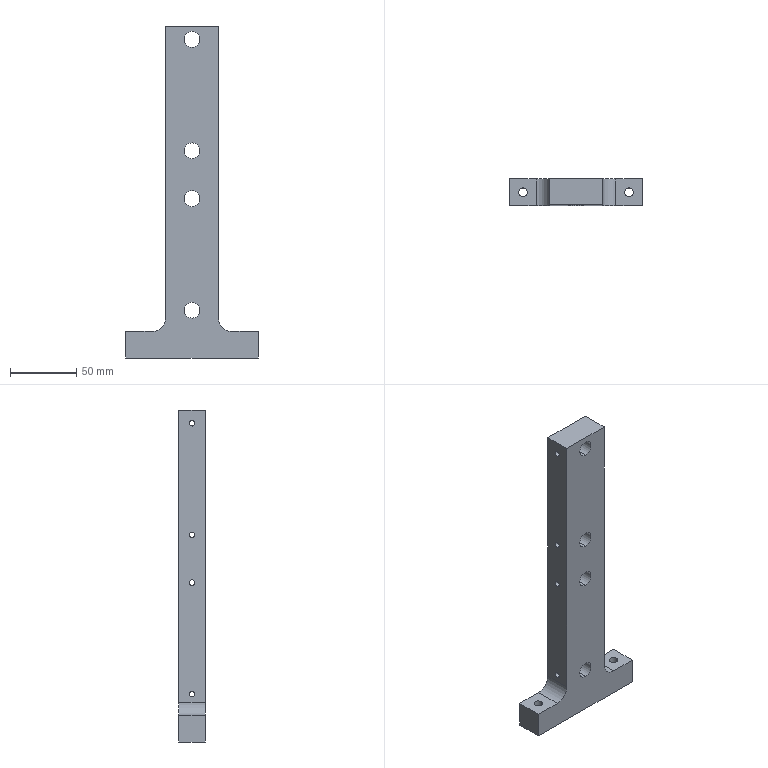Component | SolidWorks | JL001-05-01-001-1 | 1 solid | 40 faces | box 100 x 20 x 250 mm | volume 212921 mm3 | cylinder 30 | plane 10 | commonest cylinder face diameters 4.2 x16 12 x8 6.5 x4 20 x2
build123d program:
from build123d import *

# Parameters (mm, degrees)
SKETCH1_W                  = 40
SKETCH1_H                  = 230
BOSS_EXTRUDE1_DEPTH        = 10
SKETCH2_W                  = 100
SKETCH2_H                  = 20
BOSS_EXTRUDE2_DEPTH        = 20
FILLET1_R                  = 10
SIZE_MM_DOWEL_PIN_HOLE1_D  = 12
F_6_5_6_5_DIAMETER_HOLE1_D = 6.5
M5_TAPPED_HOLE1_D          = 4.2


with BuildPart() as part:
    # Sketch1 → Boss-Extrude1 (new, symmetric)
    with BuildSketch(Plane(origin=(0, 0, 0), x_dir=(1, 0, 0), z_dir=(0, 1, 0))):
        Rectangle(SKETCH1_W, SKETCH1_H)
    extrude(amount=BOSS_EXTRUDE1_DEPTH, both=True)

    # Sketch2 → Boss-Extrude2 (add)
    with BuildSketch(Plane(origin=(0, 0, -115), x_dir=(-1, 0, 0), z_dir=(0, 0, -1))):
        Rectangle(SKETCH2_W, SKETCH2_H)
    extrude(amount=BOSS_EXTRUDE2_DEPTH)

    # Fillet1
    fillet1_edges = [part.edges().sort_by_distance(p)[0] for p in [
        (-20, 0, -115),
        (20, 0, -115),
    ]]
    fillet(fillet1_edges, radius=FILLET1_R)

    # Size mm Dowel Pin Hole1 (through all)
    with Locations(Plane(origin=(0, 10, 0), x_dir=(1, 0, 0), z_dir=(0, 1, 0))):
        with Locations((0, -105), (0, 99), (0, -21), (0, 15)):
            Hole(SIZE_MM_DOWEL_PIN_HOLE1_D / 2)

    # 6.5 _6.5_ Diameter Hole1 (through all)
    with Locations(Plane.XY.offset(-115)):
        with Locations((-40, 0), (40, 0)):
            Hole(F_6_5_6_5_DIAMETER_HOLE1_D / 2)

    # M5 Tapped Hole1 (through all)
    with Locations(Plane(origin=(20, 0, 0), x_dir=(0, 0, -1), z_dir=(1, 0, 0))):
        with Locations((-105, 0), (-21, 0), (15, 0), (99, 0)):
            Hole(M5_TAPPED_HOLE1_D / 2)


solid = part.part